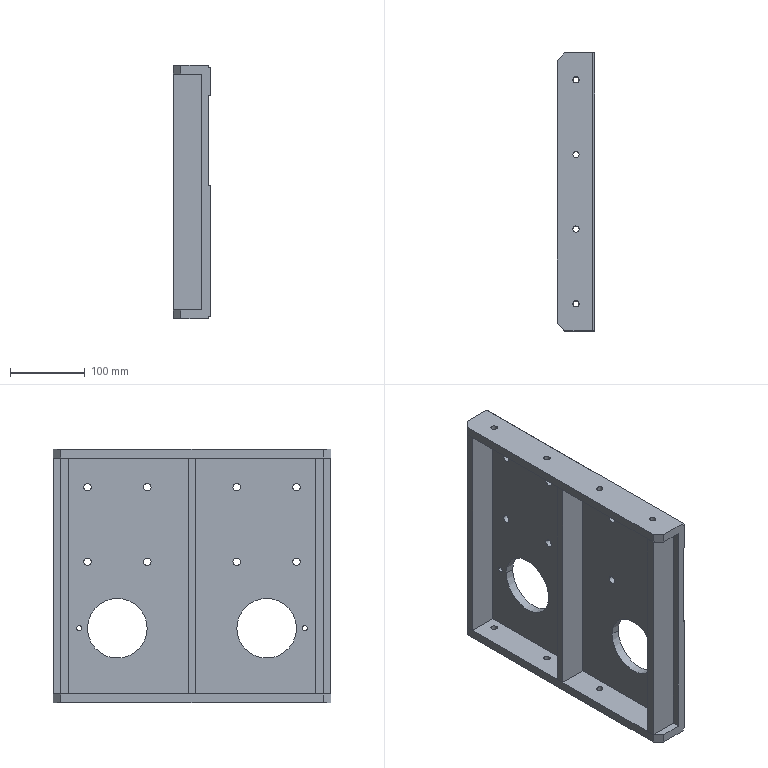Component | SolidWorks | MovingVerticalPlate1-1 | 4 solids | 80 faces | volume 1941408 mm3 | plane 40 | cylinder 40 | commonest cylinder face diameters 10.2 x16 8.5 x16 6.8 x4 80 x4